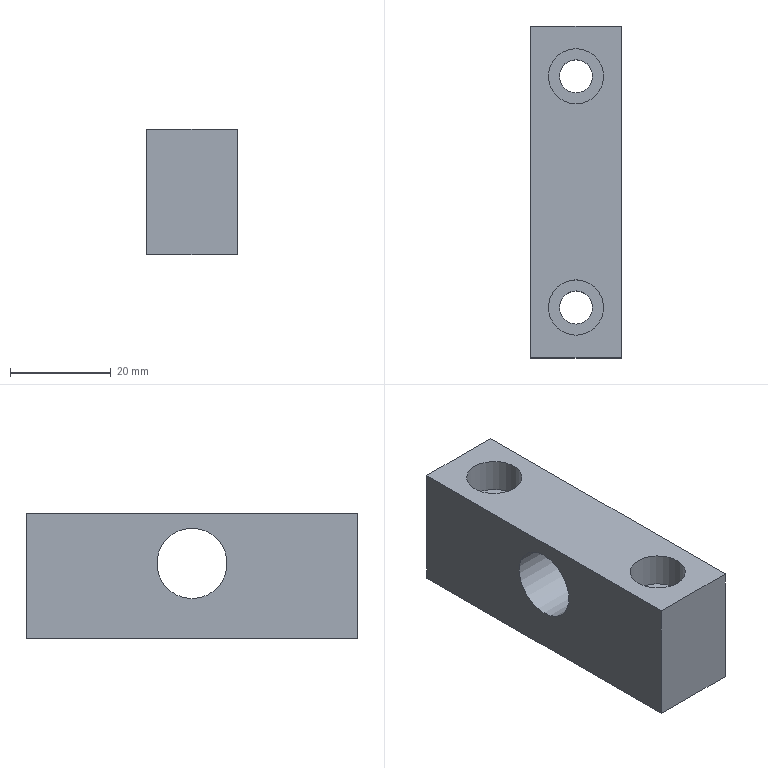Component | NX | FIXED_BLOCK | 1 solid | 13 faces | box 18 x 66 x 25 mm | volume 24391 mm3 | plane 8 | cylinder 5 | commonest cylinder face diameters 6.6 x2 11 x2 14 x1
STEP:
#1=CARTESIAN_POINT('',(0.,0.,0.));
#2=DIRECTION('',(0.,0.,1.));
#3=DIRECTION('',(1.,0.,0.));
#4=AXIS2_PLACEMENT_3D('',#1,#2,#3);
#5=CARTESIAN_POINT('',(-140.,-33.,25.));
#6=VERTEX_POINT('',#5);
#7=CARTESIAN_POINT('',(-122.,-33.,25.));
#8=VERTEX_POINT('',#7);
#9=CARTESIAN_POINT('',(-140.,-33.,25.));
#10=DIRECTION('',(1.,0.,0.));
#11=VECTOR('',#10,1.);
#12=LINE('',#9,#11);
#13=CARTESIAN_POINT('',(-140.,-33.,0.));
#14=DIRECTION('',(0.,-1.,0.));
#15=DIRECTION('',(0.,0.,1.));
#16=AXIS2_PLACEMENT_3D('',#13,#14,#15);
#17=PLANE('',#16);
#18=CARTESIAN_POINT('',(25.,0.));
#19=DIRECTION('',(0.,-1.));
#20=VECTOR('',#19,1.);
#21=LINE('',#18,#20);
#22=(GEOMETRIC_REPRESENTATION_CONTEXT(2)PARAMETRIC_REPRESENTATION_CONTEXT()REPRESENTATION_CONTEXT('',''));
#23=DEFINITIONAL_REPRESENTATION('',(#21),#22);
#24=PCURVE('',#17,#23);
#25=CARTESIAN_POINT('',(-131.,0.,25.));
#26=DIRECTION('',(0.,0.,1.));
#27=DIRECTION('',(0.,1.,0.));
#28=AXIS2_PLACEMENT_3D('',#25,#26,#27);
#29=PLANE('',#28);
#30=CARTESIAN_POINT('',(-33.,9.));
#31=DIRECTION('',(0.,-1.));
#32=VECTOR('',#31,1.);
#33=LINE('',#30,#32);
#34=(GEOMETRIC_REPRESENTATION_CONTEXT(2)PARAMETRIC_REPRESENTATION_CONTEXT()REPRESENTATION_CONTEXT('',''));
#35=DEFINITIONAL_REPRESENTATION('',(#33),#34);
#36=PCURVE('',#29,#35);
#37=SURFACE_CURVE('',#12,(#24,#36),.PCURVE_S1.);
#38=EDGE_CURVE('',#6,#8,#37,.T.);
#39=ORIENTED_EDGE('',*,*,#38,.F.);
#40=CARTESIAN_POINT('',(-140.,-33.,0.));
#41=VERTEX_POINT('',#40);
#42=CARTESIAN_POINT('',(-140.,-33.,0.));
#43=DIRECTION('',(0.,0.,1.));
#44=VECTOR('',#43,1.);
#45=LINE('',#42,#44);
#46=CARTESIAN_POINT('',(0.,0.));
#47=DIRECTION('',(1.,0.));
#48=VECTOR('',#47,1.);
#49=LINE('',#46,#48);
#50=(GEOMETRIC_REPRESENTATION_CONTEXT(2)PARAMETRIC_REPRESENTATION_CONTEXT()REPRESENTATION_CONTEXT('',''));
#51=DEFINITIONAL_REPRESENTATION('',(#49),#50);
#52=PCURVE('',#17,#51);
#53=CARTESIAN_POINT('',(-140.,33.,0.));
#54=DIRECTION('',(-1.,0.,0.));
#55=DIRECTION('',(0.,0.,1.));
#56=AXIS2_PLACEMENT_3D('',#53,#54,#55);
#57=PLANE('',#56);
#58=CARTESIAN_POINT('',(0.,-66.));
#59=DIRECTION('',(1.,0.));
#60=VECTOR('',#59,1.);
#61=LINE('',#58,#60);
#62=(GEOMETRIC_REPRESENTATION_CONTEXT(2)PARAMETRIC_REPRESENTATION_CONTEXT()REPRESENTATION_CONTEXT('',''));
#63=DEFINITIONAL_REPRESENTATION('',(#61),#62);
#64=PCURVE('',#57,#63);
#65=SURFACE_CURVE('',#45,(#52,#64),.PCURVE_S1.);
#66=EDGE_CURVE('',#41,#6,#65,.T.);
#67=ORIENTED_EDGE('',*,*,#66,.F.);
#68=CARTESIAN_POINT('',(-122.,-33.,0.));
#69=VERTEX_POINT('',#68);
#70=CARTESIAN_POINT('',(-140.,-33.,0.));
#71=DIRECTION('',(1.,0.,0.));
#72=VECTOR('',#71,1.);
#73=LINE('',#70,#72);
#74=CARTESIAN_POINT('',(0.,0.));
#75=DIRECTION('',(0.,-1.));
#76=VECTOR('',#75,1.);
#77=LINE('',#74,#76);
#78=(GEOMETRIC_REPRESENTATION_CONTEXT(2)PARAMETRIC_REPRESENTATION_CONTEXT()REPRESENTATION_CONTEXT('',''));
#79=DEFINITIONAL_REPRESENTATION('',(#77),#78);
#80=PCURVE('',#17,#79);
#81=CARTESIAN_POINT('',(-131.,0.,0.));
#82=DIRECTION('',(0.,0.,1.));
#83=DIRECTION('',(0.,1.,0.));
#84=AXIS2_PLACEMENT_3D('',#81,#82,#83);
#85=PLANE('',#84);
#86=CARTESIAN_POINT('',(-33.,9.));
#87=DIRECTION('',(0.,-1.));
#88=VECTOR('',#87,1.);
#89=LINE('',#86,#88);
#90=(GEOMETRIC_REPRESENTATION_CONTEXT(2)PARAMETRIC_REPRESENTATION_CONTEXT()REPRESENTATION_CONTEXT('',''));
#91=DEFINITIONAL_REPRESENTATION('',(#89),#90);
#92=PCURVE('',#85,#91);
#93=SURFACE_CURVE('',#73,(#80,#92),.PCURVE_S1.);
#94=EDGE_CURVE('',#41,#69,#93,.T.);
#95=ORIENTED_EDGE('',*,*,#94,.T.);
#96=CARTESIAN_POINT('',(-122.,-33.,0.));
#97=DIRECTION('',(0.,0.,1.));
#98=VECTOR('',#97,1.);
#99=LINE('',#96,#98);
#100=CARTESIAN_POINT('',(0.,-18.));
#101=DIRECTION('',(1.,0.));
#102=VECTOR('',#101,1.);
#103=LINE('',#100,#102);
#104=(GEOMETRIC_REPRESENTATION_CONTEXT(2)PARAMETRIC_REPRESENTATION_CONTEXT()REPRESENTATION_CONTEXT('',''));
#105=DEFINITIONAL_REPRESENTATION('',(#103),#104);
#106=PCURVE('',#17,#105);
#107=CARTESIAN_POINT('',(-122.,-33.,0.));
#108=DIRECTION('',(1.,0.,0.));
#109=DIRECTION('',(0.,0.,-1.));
#110=AXIS2_PLACEMENT_3D('',#107,#108,#109);
#111=PLANE('',#110);
#112=CARTESIAN_POINT('',(0.,0.));
#113=DIRECTION('',(-1.,0.));
#114=VECTOR('',#113,1.);
#115=LINE('',#112,#114);
#116=(GEOMETRIC_REPRESENTATION_CONTEXT(2)PARAMETRIC_REPRESENTATION_CONTEXT()REPRESENTATION_CONTEXT('',''));
#117=DEFINITIONAL_REPRESENTATION('',(#115),#116);
#118=PCURVE('',#111,#117);
#119=SURFACE_CURVE('',#99,(#106,#118),.PCURVE_S1.);
#120=EDGE_CURVE('',#69,#8,#119,.T.);
#121=ORIENTED_EDGE('',*,*,#120,.T.);
#122=EDGE_LOOP('',(#39,#67,#95,#121));
#123=FACE_BOUND('',#122,.T.);
#124=ADVANCED_FACE('',(#123),#17,.T.);
#125=CARTESIAN_POINT('',(-122.,0.,8.));
#126=VERTEX_POINT('',#125);
#127=CARTESIAN_POINT('',(-122.,0.,15.));
#128=DIRECTION('',(1.,0.,0.));
#129=DIRECTION('',(0.,0.,-1.));
#130=AXIS2_PLACEMENT_3D('',#127,#128,#129);
#131=CIRCLE('',#130,7.);
#132=CARTESIAN_POINT('',(-15.,33.));
#133=DIRECTION('',(1.,0.));
#134=AXIS2_PLACEMENT_2D('',#132,#133);
#135=CIRCLE('',#134,7.);
#136=(GEOMETRIC_REPRESENTATION_CONTEXT(2)PARAMETRIC_REPRESENTATION_CONTEXT()REPRESENTATION_CONTEXT('',''));
#137=DEFINITIONAL_REPRESENTATION('',(#135),#136);
#138=PCURVE('',#111,#137);
#139=CARTESIAN_POINT('',(-121.,0.,15.));
#140=DIRECTION('',(-1.,0.,0.));
#141=DIRECTION('',(0.,1.,0.));
#142=AXIS2_PLACEMENT_3D('',#139,#140,#141);
#143=CYLINDRICAL_SURFACE('',#142,7.);
#144=CARTESIAN_POINT('',(7.854,1.));
#145=DIRECTION('',(-1.,0.));
#146=VECTOR('',#145,1.);
#147=LINE('',#144,#146);
#148=(GEOMETRIC_REPRESENTATION_CONTEXT(2)PARAMETRIC_REPRESENTATION_CONTEXT()REPRESENTATION_CONTEXT('',''));
#149=DEFINITIONAL_REPRESENTATION('',(#147),#148);
#150=PCURVE('',#143,#149);
#151=SURFACE_CURVE('',#131,(#138,#150),.PCURVE_S1.);
#152=EDGE_CURVE('',#126,#126,#151,.T.);
#153=ORIENTED_EDGE('',*,*,#152,.F.);
#154=EDGE_LOOP('',(#153));
#155=FACE_BOUND('',#154,.T.);
#156=CARTESIAN_POINT('',(-122.,33.,25.));
#157=VERTEX_POINT('',#156);
#158=CARTESIAN_POINT('',(-122.,-33.,25.));
#159=DIRECTION('',(0.,1.,0.));
#160=VECTOR('',#159,1.);
#161=LINE('',#158,#160);
#162=CARTESIAN_POINT('',(-25.,0.));
#163=DIRECTION('',(0.,1.));
#164=VECTOR('',#163,1.);
#165=LINE('',#162,#164);
#166=(GEOMETRIC_REPRESENTATION_CONTEXT(2)PARAMETRIC_REPRESENTATION_CONTEXT()REPRESENTATION_CONTEXT('',''));
#167=DEFINITIONAL_REPRESENTATION('',(#165),#166);
#168=PCURVE('',#111,#167);
#169=CARTESIAN_POINT('',(-33.,-9.));
#170=DIRECTION('',(1.,0.));
#171=VECTOR('',#170,1.);
#172=LINE('',#169,#171);
#173=(GEOMETRIC_REPRESENTATION_CONTEXT(2)PARAMETRIC_REPRESENTATION_CONTEXT()REPRESENTATION_CONTEXT('',''));
#174=DEFINITIONAL_REPRESENTATION('',(#172),#173);
#175=PCURVE('',#29,#174);
#176=SURFACE_CURVE('',#161,(#168,#175),.PCURVE_S1.);
#177=EDGE_CURVE('',#8,#157,#176,.T.);
#178=ORIENTED_EDGE('',*,*,#177,.F.);
#179=ORIENTED_EDGE('',*,*,#120,.F.);
#180=CARTESIAN_POINT('',(-122.,33.,0.));
#181=VERTEX_POINT('',#180);
#182=CARTESIAN_POINT('',(-122.,-33.,0.));
#183=DIRECTION('',(0.,1.,0.));
#184=VECTOR('',#183,1.);
#185=LINE('',#182,#184);
#186=CARTESIAN_POINT('',(0.,0.));
#187=DIRECTION('',(0.,1.));
#188=VECTOR('',#187,1.);
#189=LINE('',#186,#188);
#190=(GEOMETRIC_REPRESENTATION_CONTEXT(2)PARAMETRIC_REPRESENTATION_CONTEXT()REPRESENTATION_CONTEXT('',''));
#191=DEFINITIONAL_REPRESENTATION('',(#189),#190);
#192=PCURVE('',#111,#191);
#193=CARTESIAN_POINT('',(-33.,-9.));
#194=DIRECTION('',(1.,0.));
#195=VECTOR('',#194,1.);
#196=LINE('',#193,#195);
#197=(GEOMETRIC_REPRESENTATION_CONTEXT(2)PARAMETRIC_REPRESENTATION_CONTEXT()REPRESENTATION_CONTEXT('',''));
#198=DEFINITIONAL_REPRESENTATION('',(#196),#197);
#199=PCURVE('',#85,#198);
#200=SURFACE_CURVE('',#185,(#192,#199),.PCURVE_S1.);
#201=EDGE_CURVE('',#69,#181,#200,.T.);
#202=ORIENTED_EDGE('',*,*,#201,.T.);
#203=CARTESIAN_POINT('',(-122.,33.,0.));
#204=DIRECTION('',(0.,0.,1.));
#205=VECTOR('',#204,1.);
#206=LINE('',#203,#205);
#207=CARTESIAN_POINT('',(0.,66.));
#208=DIRECTION('',(-1.,0.));
#209=VECTOR('',#208,1.);
#210=LINE('',#207,#209);
#211=(GEOMETRIC_REPRESENTATION_CONTEXT(2)PARAMETRIC_REPRESENTATION_CONTEXT()REPRESENTATION_CONTEXT('',''));
#212=DEFINITIONAL_REPRESENTATION('',(#210),#211);
#213=PCURVE('',#111,#212);
#214=CARTESIAN_POINT('',(-122.,33.,0.));
#215=DIRECTION('',(0.,1.,0.));
#216=DIRECTION('',(0.,0.,-1.));
#217=AXIS2_PLACEMENT_3D('',#214,#215,#216);
#218=PLANE('',#217);
#219=CARTESIAN_POINT('',(0.,0.));
#220=DIRECTION('',(-1.,0.));
#221=VECTOR('',#220,1.);
#222=LINE('',#219,#221);
#223=(GEOMETRIC_REPRESENTATION_CONTEXT(2)PARAMETRIC_REPRESENTATION_CONTEXT()REPRESENTATION_CONTEXT('',''));
#224=DEFINITIONAL_REPRESENTATION('',(#222),#223);
#225=PCURVE('',#218,#224);
#226=SURFACE_CURVE('',#206,(#213,#225),.PCURVE_S1.);
#227=EDGE_CURVE('',#181,#157,#226,.T.);
#228=ORIENTED_EDGE('',*,*,#227,.T.);
#229=EDGE_LOOP('',(#178,#179,#202,#228));
#230=FACE_BOUND('',#229,.T.);
#231=ADVANCED_FACE('',(#155,#230),#111,.T.);
#232=CARTESIAN_POINT('',(-140.,33.,25.));
#233=VERTEX_POINT('',#232);
#234=CARTESIAN_POINT('',(-122.,33.,25.));
#235=DIRECTION('',(-1.,0.,0.));
#236=VECTOR('',#235,1.);
#237=LINE('',#234,#236);
#238=CARTESIAN_POINT('',(-25.,0.));
#239=DIRECTION('',(0.,1.));
#240=VECTOR('',#239,1.);
#241=LINE('',#238,#240);
#242=(GEOMETRIC_REPRESENTATION_CONTEXT(2)PARAMETRIC_REPRESENTATION_CONTEXT()REPRESENTATION_CONTEXT('',''));
#243=DEFINITIONAL_REPRESENTATION('',(#241),#242);
#244=PCURVE('',#218,#243);
#245=CARTESIAN_POINT('',(33.,-9.));
#246=DIRECTION('',(0.,1.));
#247=VECTOR('',#246,1.);
#248=LINE('',#245,#247);
#249=(GEOMETRIC_REPRESENTATION_CONTEXT(2)PARAMETRIC_REPRESENTATION_CONTEXT()REPRESENTATION_CONTEXT('',''));
#250=DEFINITIONAL_REPRESENTATION('',(#248),#249);
#251=PCURVE('',#29,#250);
#252=SURFACE_CURVE('',#237,(#244,#251),.PCURVE_S1.);
#253=EDGE_CURVE('',#157,#233,#252,.T.);
#254=ORIENTED_EDGE('',*,*,#253,.F.);
#255=ORIENTED_EDGE('',*,*,#227,.F.);
#256=CARTESIAN_POINT('',(-140.,33.,0.));
#257=VERTEX_POINT('',#256);
#258=CARTESIAN_POINT('',(-122.,33.,0.));
#259=DIRECTION('',(-1.,0.,0.));
#260=VECTOR('',#259,1.);
#261=LINE('',#258,#260);
#262=CARTESIAN_POINT('',(0.,0.));
#263=DIRECTION('',(0.,1.));
#264=VECTOR('',#263,1.);
#265=LINE('',#262,#264);
#266=(GEOMETRIC_REPRESENTATION_CONTEXT(2)PARAMETRIC_REPRESENTATION_CONTEXT()REPRESENTATION_CONTEXT('',''));
#267=DEFINITIONAL_REPRESENTATION('',(#265),#266);
#268=PCURVE('',#218,#267);
#269=CARTESIAN_POINT('',(33.,-9.));
#270=DIRECTION('',(0.,1.));
#271=VECTOR('',#270,1.);
#272=LINE('',#269,#271);
#273=(GEOMETRIC_REPRESENTATION_CONTEXT(2)PARAMETRIC_REPRESENTATION_CONTEXT()REPRESENTATION_CONTEXT('',''));
#274=DEFINITIONAL_REPRESENTATION('',(#272),#273);
#275=PCURVE('',#85,#274);
#276=SURFACE_CURVE('',#261,(#268,#275),.PCURVE_S1.);
#277=EDGE_CURVE('',#181,#257,#276,.T.);
#278=ORIENTED_EDGE('',*,*,#277,.T.);
#279=CARTESIAN_POINT('',(-140.,33.,0.));
#280=DIRECTION('',(0.,0.,1.));
#281=VECTOR('',#280,1.);
#282=LINE('',#279,#281);
#283=CARTESIAN_POINT('',(0.,18.));
#284=DIRECTION('',(-1.,0.));
#285=VECTOR('',#284,1.);
#286=LINE('',#283,#285);
#287=(GEOMETRIC_REPRESENTATION_CONTEXT(2)PARAMETRIC_REPRESENTATION_CONTEXT()REPRESENTATION_CONTEXT('',''));
#288=DEFINITIONAL_REPRESENTATION('',(#286),#287);
#289=PCURVE('',#218,#288);
#290=CARTESIAN_POINT('',(0.,0.));
#291=DIRECTION('',(1.,0.));
#292=VECTOR('',#291,1.);
#293=LINE('',#290,#292);
#294=(GEOMETRIC_REPRESENTATION_CONTEXT(2)PARAMETRIC_REPRESENTATION_CONTEXT()REPRESENTATION_CONTEXT('',''));
#295=DEFINITIONAL_REPRESENTATION('',(#293),#294);
#296=PCURVE('',#57,#295);
#297=SURFACE_CURVE('',#282,(#289,#296),.PCURVE_S1.);
#298=EDGE_CURVE('',#257,#233,#297,.T.);
#299=ORIENTED_EDGE('',*,*,#298,.T.);
#300=EDGE_LOOP('',(#254,#255,#278,#299));
#301=FACE_BOUND('',#300,.T.);
#302=ADVANCED_FACE('',(#301),#218,.T.);
#303=CARTESIAN_POINT('',(-140.,0.,22.));
#304=VERTEX_POINT('',#303);
#305=CARTESIAN_POINT('',(-140.,0.,8.));
#306=VERTEX_POINT('',#305);
#307=CARTESIAN_POINT('',(-140.,0.,15.));
#308=DIRECTION('',(-1.,0.,0.));
#309=DIRECTION('',(0.,0.,1.));
#310=AXIS2_PLACEMENT_3D('',#307,#308,#309);
#311=CIRCLE('',#310,7.);
#312=CARTESIAN_POINT('',(15.,-33.));
#313=DIRECTION('',(1.,0.));
#314=AXIS2_PLACEMENT_2D('',#312,#313);
#315=CIRCLE('',#314,7.);
#316=(GEOMETRIC_REPRESENTATION_CONTEXT(2)PARAMETRIC_REPRESENTATION_CONTEXT()REPRESENTATION_CONTEXT('',''));
#317=DEFINITIONAL_REPRESENTATION('',(#315),#316);
#318=PCURVE('',#57,#317);
#319=CARTESIAN_POINT('',(4.712,19.));
#320=DIRECTION('',(1.,0.));
#321=VECTOR('',#320,1.);
#322=LINE('',#319,#321);
#323=(GEOMETRIC_REPRESENTATION_CONTEXT(2)PARAMETRIC_REPRESENTATION_CONTEXT()REPRESENTATION_CONTEXT('',''));
#324=DEFINITIONAL_REPRESENTATION('',(#322),#323);
#325=PCURVE('',#143,#324);
#326=SURFACE_CURVE('',#311,(#318,#325),.PCURVE_S1.);
#327=EDGE_CURVE('',#304,#306,#326,.T.);
#328=ORIENTED_EDGE('',*,*,#327,.F.);
#329=CARTESIAN_POINT('',(-140.,0.,15.));
#330=DIRECTION('',(-1.,0.,0.));
#331=DIRECTION('',(0.,0.,1.));
#332=AXIS2_PLACEMENT_3D('',#329,#330,#331);
#333=CIRCLE('',#332,7.);
#334=CARTESIAN_POINT('',(15.,-33.));
#335=DIRECTION('',(1.,0.));
#336=AXIS2_PLACEMENT_2D('',#334,#335);
#337=CIRCLE('',#336,7.);
#338=(GEOMETRIC_REPRESENTATION_CONTEXT(2)PARAMETRIC_REPRESENTATION_CONTEXT()REPRESENTATION_CONTEXT('',''));
#339=DEFINITIONAL_REPRESENTATION('',(#337),#338);
#340=PCURVE('',#57,#339);
#341=CARTESIAN_POINT('',(-1.571,19.));
#342=DIRECTION('',(1.,0.));
#343=VECTOR('',#342,1.);
#344=LINE('',#341,#343);
#345=(GEOMETRIC_REPRESENTATION_CONTEXT(2)PARAMETRIC_REPRESENTATION_CONTEXT()REPRESENTATION_CONTEXT('',''));
#346=DEFINITIONAL_REPRESENTATION('',(#344),#345);
#347=PCURVE('',#143,#346);
#348=SURFACE_CURVE('',#333,(#340,#347),.PCURVE_S1.);
#349=EDGE_CURVE('',#306,#304,#348,.T.);
#350=ORIENTED_EDGE('',*,*,#349,.F.);
#351=EDGE_LOOP('',(#328,#350));
#352=FACE_BOUND('',#351,.T.);
#353=CARTESIAN_POINT('',(-140.,33.,25.));
#354=DIRECTION('',(0.,-1.,0.));
#355=VECTOR('',#354,1.);
#356=LINE('',#353,#355);
#357=CARTESIAN_POINT('',(25.,0.));
#358=DIRECTION('',(0.,-1.));
#359=VECTOR('',#358,1.);
#360=LINE('',#357,#359);
#361=(GEOMETRIC_REPRESENTATION_CONTEXT(2)PARAMETRIC_REPRESENTATION_CONTEXT()REPRESENTATION_CONTEXT('',''));
#362=DEFINITIONAL_REPRESENTATION('',(#360),#361);
#363=PCURVE('',#57,#362);
#364=CARTESIAN_POINT('',(33.,9.));
#365=DIRECTION('',(-1.,0.));
#366=VECTOR('',#365,1.);
#367=LINE('',#364,#366);
#368=(GEOMETRIC_REPRESENTATION_CONTEXT(2)PARAMETRIC_REPRESENTATION_CONTEXT()REPRESENTATION_CONTEXT('',''));
#369=DEFINITIONAL_REPRESENTATION('',(#367),#368);
#370=PCURVE('',#29,#369);
#371=SURFACE_CURVE('',#356,(#363,#370),.PCURVE_S1.);
#372=EDGE_CURVE('',#233,#6,#371,.T.);
#373=ORIENTED_EDGE('',*,*,#372,.F.);
#374=ORIENTED_EDGE('',*,*,#298,.F.);
#375=CARTESIAN_POINT('',(-140.,33.,0.));
#376=DIRECTION('',(0.,-1.,0.));
#377=VECTOR('',#376,1.);
#378=LINE('',#375,#377);
#379=CARTESIAN_POINT('',(0.,0.));
#380=DIRECTION('',(0.,-1.));
#381=VECTOR('',#380,1.);
#382=LINE('',#379,#381);
#383=(GEOMETRIC_REPRESENTATION_CONTEXT(2)PARAMETRIC_REPRESENTATION_CONTEXT()REPRESENTATION_CONTEXT('',''));
#384=DEFINITIONAL_REPRESENTATION('',(#382),#383);
#385=PCURVE('',#57,#384);
#386=CARTESIAN_POINT('',(33.,9.));
#387=DIRECTION('',(-1.,0.));
#388=VECTOR('',#387,1.);
#389=LINE('',#386,#388);
#390=(GEOMETRIC_REPRESENTATION_CONTEXT(2)PARAMETRIC_REPRESENTATION_CONTEXT()REPRESENTATION_CONTEXT('',''));
#391=DEFINITIONAL_REPRESENTATION('',(#389),#390);
#392=PCURVE('',#85,#391);
#393=SURFACE_CURVE('',#378,(#385,#392),.PCURVE_S1.);
#394=EDGE_CURVE('',#257,#41,#393,.T.);
#395=ORIENTED_EDGE('',*,*,#394,.T.);
#396=ORIENTED_EDGE('',*,*,#66,.T.);
#397=EDGE_LOOP('',(#373,#374,#395,#396));
#398=FACE_BOUND('',#397,.T.);
#399=ADVANCED_FACE('',(#352,#398),#57,.T.);
#400=CARTESIAN_POINT('',(-131.,26.3,0.));
#401=VERTEX_POINT('',#400);
#402=CARTESIAN_POINT('',(-131.,19.7,0.));
#403=VERTEX_POINT('',#402);
#404=CARTESIAN_POINT('',(-131.,23.,0.));
#405=DIRECTION('',(0.,0.,1.));
#406=DIRECTION('',(0.,1.,0.));
#407=AXIS2_PLACEMENT_3D('',#404,#405,#406);
#408=CIRCLE('',#407,3.3);
#409=CARTESIAN_POINT('',(23.,0.));
#410=DIRECTION('',(1.,0.));
#411=AXIS2_PLACEMENT_2D('',#409,#410);
#412=CIRCLE('',#411,3.3);
#413=(GEOMETRIC_REPRESENTATION_CONTEXT(2)PARAMETRIC_REPRESENTATION_CONTEXT()REPRESENTATION_CONTEXT('',''));
#414=DEFINITIONAL_REPRESENTATION('',(#412),#413);
#415=PCURVE('',#85,#414);
#416=CARTESIAN_POINT('',(-131.,23.,-20.299));
#417=DIRECTION('',(0.,0.,-1.));
#418=DIRECTION('',(0.,-1.,0.));
#419=AXIS2_PLACEMENT_3D('',#416,#417,#418);
#420=CYLINDRICAL_SURFACE('',#419,3.3);
#421=CARTESIAN_POINT('',(3.142,-20.299));
#422=DIRECTION('',(-1.,0.));
#423=VECTOR('',#422,1.);
#424=LINE('',#421,#423);
#425=(GEOMETRIC_REPRESENTATION_CONTEXT(2)PARAMETRIC_REPRESENTATION_CONTEXT()REPRESENTATION_CONTEXT('',''));
#426=DEFINITIONAL_REPRESENTATION('',(#424),#425);
#427=PCURVE('',#420,#426);
#428=SURFACE_CURVE('',#408,(#415,#427),.PCURVE_S1.);
#429=EDGE_CURVE('',#401,#403,#428,.T.);
#430=ORIENTED_EDGE('',*,*,#429,.T.);
#431=CARTESIAN_POINT('',(-131.,23.,0.));
#432=DIRECTION('',(0.,0.,1.));
#433=DIRECTION('',(0.,1.,0.));
#434=AXIS2_PLACEMENT_3D('',#431,#432,#433);
#435=CIRCLE('',#434,3.3);
#436=CARTESIAN_POINT('',(23.,0.));
#437=DIRECTION('',(1.,0.));
#438=AXIS2_PLACEMENT_2D('',#436,#437);
#439=CIRCLE('',#438,3.3);
#440=(GEOMETRIC_REPRESENTATION_CONTEXT(2)PARAMETRIC_REPRESENTATION_CONTEXT()REPRESENTATION_CONTEXT('',''));
#441=DEFINITIONAL_REPRESENTATION('',(#439),#440);
#442=PCURVE('',#85,#441);
#443=CARTESIAN_POINT('',(9.425,-20.299));
#444=DIRECTION('',(-1.,0.));
#445=VECTOR('',#444,1.);
#446=LINE('',#443,#445);
#447=(GEOMETRIC_REPRESENTATION_CONTEXT(2)PARAMETRIC_REPRESENTATION_CONTEXT()REPRESENTATION_CONTEXT('',''));
#448=DEFINITIONAL_REPRESENTATION('',(#446),#447);
#449=PCURVE('',#420,#448);
#450=SURFACE_CURVE('',#435,(#442,#449),.PCURVE_S1.);
#451=EDGE_CURVE('',#403,#401,#450,.T.);
#452=ORIENTED_EDGE('',*,*,#451,.T.);
#453=EDGE_LOOP('',(#430,#452));
#454=FACE_BOUND('',#453,.T.);
#455=CARTESIAN_POINT('',(-131.,-19.7,0.));
#456=VERTEX_POINT('',#455);
#457=CARTESIAN_POINT('',(-131.,-26.3,0.));
#458=VERTEX_POINT('',#457);
#459=CARTESIAN_POINT('',(-131.,-23.,0.));
#460=DIRECTION('',(0.,0.,1.));
#461=DIRECTION('',(0.,1.,0.));
#462=AXIS2_PLACEMENT_3D('',#459,#460,#461);
#463=CIRCLE('',#462,3.3);
#464=CARTESIAN_POINT('',(-23.,0.));
#465=DIRECTION('',(1.,0.));
#466=AXIS2_PLACEMENT_2D('',#464,#465);
#467=CIRCLE('',#466,3.3);
#468=(GEOMETRIC_REPRESENTATION_CONTEXT(2)PARAMETRIC_REPRESENTATION_CONTEXT()REPRESENTATION_CONTEXT('',''));
#469=DEFINITIONAL_REPRESENTATION('',(#467),#468);
#470=PCURVE('',#85,#469);
#471=CARTESIAN_POINT('',(-131.,-23.,-20.299));
#472=DIRECTION('',(0.,0.,-1.));
#473=DIRECTION('',(0.,-1.,0.));
#474=AXIS2_PLACEMENT_3D('',#471,#472,#473);
#475=CYLINDRICAL_SURFACE('',#474,3.3);
#476=CARTESIAN_POINT('',(3.142,-20.299));
#477=DIRECTION('',(-1.,0.));
#478=VECTOR('',#477,1.);
#479=LINE('',#476,#478);
#480=(GEOMETRIC_REPRESENTATION_CONTEXT(2)PARAMETRIC_REPRESENTATION_CONTEXT()REPRESENTATION_CONTEXT('',''));
#481=DEFINITIONAL_REPRESENTATION('',(#479),#480);
#482=PCURVE('',#475,#481);
#483=SURFACE_CURVE('',#463,(#470,#482),.PCURVE_S1.);
#484=EDGE_CURVE('',#456,#458,#483,.T.);
#485=ORIENTED_EDGE('',*,*,#484,.T.);
#486=CARTESIAN_POINT('',(-131.,-23.,0.));
#487=DIRECTION('',(0.,0.,1.));
#488=DIRECTION('',(0.,1.,0.));
#489=AXIS2_PLACEMENT_3D('',#486,#487,#488);
#490=CIRCLE('',#489,3.3);
#491=CARTESIAN_POINT('',(-23.,0.));
#492=DIRECTION('',(1.,0.));
#493=AXIS2_PLACEMENT_2D('',#491,#492);
#494=CIRCLE('',#493,3.3);
#495=(GEOMETRIC_REPRESENTATION_CONTEXT(2)PARAMETRIC_REPRESENTATION_CONTEXT()REPRESENTATION_CONTEXT('',''));
#496=DEFINITIONAL_REPRESENTATION('',(#494),#495);
#497=PCURVE('',#85,#496);
#498=CARTESIAN_POINT('',(9.425,-20.299));
#499=DIRECTION('',(-1.,0.));
#500=VECTOR('',#499,1.);
#501=LINE('',#498,#500);
#502=(GEOMETRIC_REPRESENTATION_CONTEXT(2)PARAMETRIC_REPRESENTATION_CONTEXT()REPRESENTATION_CONTEXT('',''));
#503=DEFINITIONAL_REPRESENTATION('',(#501),#502);
#504=PCURVE('',#475,#503);
#505=SURFACE_CURVE('',#490,(#497,#504),.PCURVE_S1.);
#506=EDGE_CURVE('',#458,#456,#505,.T.);
#507=ORIENTED_EDGE('',*,*,#506,.T.);
#508=EDGE_LOOP('',(#485,#507));
#509=FACE_BOUND('',#508,.T.);
#510=ORIENTED_EDGE('',*,*,#94,.F.);
#511=ORIENTED_EDGE('',*,*,#394,.F.);
#512=ORIENTED_EDGE('',*,*,#277,.F.);
#513=ORIENTED_EDGE('',*,*,#201,.F.);
#514=EDGE_LOOP('',(#510,#511,#512,#513));
#515=FACE_BOUND('',#514,.T.);
#516=ADVANCED_FACE('',(#454,#509,#515),#85,.F.);
#517=CARTESIAN_POINT('',(-131.,17.5,25.));
#518=VERTEX_POINT('',#517);
#519=CARTESIAN_POINT('',(-131.,23.,25.));
#520=DIRECTION('',(0.,0.,-1.));
#521=DIRECTION('',(0.,-1.,0.));
#522=AXIS2_PLACEMENT_3D('',#519,#520,#521);
#523=CIRCLE('',#522,5.5);
#524=CARTESIAN_POINT('',(17.5,0.));
#525=CARTESIAN_POINT('',(17.5,9.526));
#526=CARTESIAN_POINT('',(25.75,4.763));
#527=CARTESIAN_POINT('',(34.,0.));
#528=CARTESIAN_POINT('',(25.75,-4.763));
#529=CARTESIAN_POINT('',(17.5,-9.526));
#530=CARTESIAN_POINT('',(17.5,0.));
#531=(BOUNDED_CURVE()B_SPLINE_CURVE(2,(#524,#525,#526,#527,#528,#529,#530),.UNSPECIFIED.,.T.,.F.)B_SPLINE_CURVE_WITH_KNOTS((1,2,2,2,2,1),(-2.094,0.,2.094,4.189,6.283,8.378),.UNSPECIFIED.)CURVE()GEOMETRIC_REPRESENTATION_ITEM()RATIONAL_B_SPLINE_CURVE((1.,0.5,1.,0.5,1.,0.5,1.))REPRESENTATION_ITEM(''));
#532=(GEOMETRIC_REPRESENTATION_CONTEXT(2)PARAMETRIC_REPRESENTATION_CONTEXT()REPRESENTATION_CONTEXT('',''));
#533=DEFINITIONAL_REPRESENTATION('',(#531),#532);
#534=PCURVE('',#29,#533);
#535=CARTESIAN_POINT('',(-131.,23.,25.));
#536=DIRECTION('',(0.,0.,-1.));
#537=DIRECTION('',(0.,-1.,0.));
#538=AXIS2_PLACEMENT_3D('',#535,#536,#537);
#539=CYLINDRICAL_SURFACE('',#538,5.5);
#540=CARTESIAN_POINT('',(0.,0.));
#541=DIRECTION('',(1.,0.));
#542=VECTOR('',#541,1.);
#543=LINE('',#540,#542);
#544=(GEOMETRIC_REPRESENTATION_CONTEXT(2)PARAMETRIC_REPRESENTATION_CONTEXT()REPRESENTATION_CONTEXT('',''));
#545=DEFINITIONAL_REPRESENTATION('',(#543),#544);
#546=PCURVE('',#539,#545);
#547=SURFACE_CURVE('',#523,(#534,#546),.PCURVE_S1.);
#548=EDGE_CURVE('',#518,#518,#547,.T.);
#549=ORIENTED_EDGE('',*,*,#548,.T.);
#550=EDGE_LOOP('',(#549));
#551=FACE_BOUND('',#550,.T.);
#552=CARTESIAN_POINT('',(-131.,-28.5,25.));
#553=VERTEX_POINT('',#552);
#554=CARTESIAN_POINT('',(-131.,-23.,25.));
#555=DIRECTION('',(0.,0.,-1.));
#556=DIRECTION('',(0.,-1.,0.));
#557=AXIS2_PLACEMENT_3D('',#554,#555,#556);
#558=CIRCLE('',#557,5.5);
#559=CARTESIAN_POINT('',(-28.5,0.));
#560=CARTESIAN_POINT('',(-28.5,9.526));
#561=CARTESIAN_POINT('',(-20.25,4.763));
#562=CARTESIAN_POINT('',(-12.,0.));
#563=CARTESIAN_POINT('',(-20.25,-4.763));
#564=CARTESIAN_POINT('',(-28.5,-9.526));
#565=CARTESIAN_POINT('',(-28.5,0.));
#566=(BOUNDED_CURVE()B_SPLINE_CURVE(2,(#559,#560,#561,#562,#563,#564,#565),.UNSPECIFIED.,.T.,.F.)B_SPLINE_CURVE_WITH_KNOTS((1,2,2,2,2,1),(-2.094,0.,2.094,4.189,6.283,8.378),.UNSPECIFIED.)CURVE()GEOMETRIC_REPRESENTATION_ITEM()RATIONAL_B_SPLINE_CURVE((1.,0.5,1.,0.5,1.,0.5,1.))REPRESENTATION_ITEM(''));
#567=(GEOMETRIC_REPRESENTATION_CONTEXT(2)PARAMETRIC_REPRESENTATION_CONTEXT()REPRESENTATION_CONTEXT('',''));
#568=DEFINITIONAL_REPRESENTATION('',(#566),#567);
#569=PCURVE('',#29,#568);
#570=CARTESIAN_POINT('',(-131.,-23.,25.));
#571=DIRECTION('',(0.,0.,-1.));
#572=DIRECTION('',(0.,-1.,0.));
#573=AXIS2_PLACEMENT_3D('',#570,#571,#572);
#574=CYLINDRICAL_SURFACE('',#573,5.5);
#575=CARTESIAN_POINT('',(0.,0.));
#576=DIRECTION('',(1.,0.));
#577=VECTOR('',#576,1.);
#578=LINE('',#575,#577);
#579=(GEOMETRIC_REPRESENTATION_CONTEXT(2)PARAMETRIC_REPRESENTATION_CONTEXT()REPRESENTATION_CONTEXT('',''));
#580=DEFINITIONAL_REPRESENTATION('',(#578),#579);
#581=PCURVE('',#574,#580);
#582=SURFACE_CURVE('',#558,(#569,#581),.PCURVE_S1.);
#583=EDGE_CURVE('',#553,#553,#582,.T.);
#584=ORIENTED_EDGE('',*,*,#583,.T.);
#585=EDGE_LOOP('',(#584));
#586=FACE_BOUND('',#585,.T.);
#587=ORIENTED_EDGE('',*,*,#38,.T.);
#588=ORIENTED_EDGE('',*,*,#177,.T.);
#589=ORIENTED_EDGE('',*,*,#253,.T.);
#590=ORIENTED_EDGE('',*,*,#372,.T.);
#591=EDGE_LOOP('',(#587,#588,#589,#590));
#592=FACE_BOUND('',#591,.T.);
#593=ADVANCED_FACE('',(#551,#586,#592),#29,.T.);
#594=CARTESIAN_POINT('',(-131.,-26.3,18.2));
#595=VERTEX_POINT('',#594);
#596=CARTESIAN_POINT('',(-131.,-23.,18.2));
#597=DIRECTION('',(0.,0.,1.));
#598=DIRECTION('',(0.,-1.,0.));
#599=AXIS2_PLACEMENT_3D('',#596,#597,#598);
#600=CIRCLE('',#599,3.3);
#601=CARTESIAN_POINT('',(6.283,-38.499));
#602=DIRECTION('',(-1.,0.));
#603=VECTOR('',#602,1.);
#604=LINE('',#601,#603);
#605=(GEOMETRIC_REPRESENTATION_CONTEXT(2)PARAMETRIC_REPRESENTATION_CONTEXT()REPRESENTATION_CONTEXT('',''));
#606=DEFINITIONAL_REPRESENTATION('',(#604),#605);
#607=PCURVE('',#475,#606);
#608=CARTESIAN_POINT('',(-131.,-23.,18.2));
#609=DIRECTION('',(0.,0.,-1.));
#610=DIRECTION('',(0.,-1.,0.));
#611=AXIS2_PLACEMENT_3D('',#608,#609,#610);
#612=PLANE('',#611);
#613=CARTESIAN_POINT('',(3.3,0.));
#614=CARTESIAN_POINT('',(3.3,-5.716));
#615=CARTESIAN_POINT('',(-1.65,-2.858));
#616=CARTESIAN_POINT('',(-6.6,-0.));
#617=CARTESIAN_POINT('',(-1.65,2.858));
#618=CARTESIAN_POINT('',(3.3,5.716));
#619=CARTESIAN_POINT('',(3.3,0.));
#620=(BOUNDED_CURVE()B_SPLINE_CURVE(2,(#613,#614,#615,#616,#617,#618,#619),.UNSPECIFIED.,.T.,.F.)B_SPLINE_CURVE_WITH_KNOTS((1,2,2,2,2,1),(-2.094,0.,2.094,4.189,6.283,8.378),.UNSPECIFIED.)CURVE()GEOMETRIC_REPRESENTATION_ITEM()RATIONAL_B_SPLINE_CURVE((1.,0.5,1.,0.5,1.,0.5,1.))REPRESENTATION_ITEM(''));
#621=(GEOMETRIC_REPRESENTATION_CONTEXT(2)PARAMETRIC_REPRESENTATION_CONTEXT()REPRESENTATION_CONTEXT('',''));
#622=DEFINITIONAL_REPRESENTATION('',(#620),#621);
#623=PCURVE('',#612,#622);
#624=SURFACE_CURVE('',#600,(#607,#623),.PCURVE_S1.);
#625=EDGE_CURVE('',#595,#595,#624,.T.);
#626=ORIENTED_EDGE('',*,*,#625,.F.);
#627=CARTESIAN_POINT('',(-131.,-26.3,18.2));
#628=CARTESIAN_POINT('',(-131.,-26.3,0.));
#629=B_SPLINE_CURVE_WITH_KNOTS('',1,(#627,#628),.UNSPECIFIED.,.F.,.F.,(2,2),(-38.499,-20.299),.PIECEWISE_BEZIER_KNOTS.);
#630=CARTESIAN_POINT('',(6.283,0.));
#631=DIRECTION('',(0.,1.));
#632=VECTOR('',#631,1.);
#633=LINE('',#630,#632);
#634=(GEOMETRIC_REPRESENTATION_CONTEXT(2)PARAMETRIC_REPRESENTATION_CONTEXT()REPRESENTATION_CONTEXT('',''));
#635=DEFINITIONAL_REPRESENTATION('',(#633),#634);
#636=PCURVE('',#475,#635);
#637=CARTESIAN_POINT('',(0.,0.));
#638=DIRECTION('',(0.,1.));
#639=VECTOR('',#638,1.);
#640=LINE('',#637,#639);
#641=(GEOMETRIC_REPRESENTATION_CONTEXT(2)PARAMETRIC_REPRESENTATION_CONTEXT()REPRESENTATION_CONTEXT('',''));
#642=DEFINITIONAL_REPRESENTATION('',(#640),#641);
#643=PCURVE('',#475,#642);
#644=SEAM_CURVE('',#629,(#636,#643),.PCURVE_S1.);
#645=EDGE_CURVE('',#595,#458,#644,.T.);
#646=ORIENTED_EDGE('',*,*,#645,.T.);
#647=ORIENTED_EDGE('',*,*,#506,.T.);
#648=ORIENTED_EDGE('',*,*,#484,.T.);
#649=ORIENTED_EDGE('',*,*,#645,.F.);
#650=EDGE_LOOP('',(#626,#646,#647,#648,#649));
#651=FACE_BOUND('',#650,.F.);
#652=ADVANCED_FACE('',(#651),#475,.F.);
#653=ORIENTED_EDGE('',*,*,#625,.F.);
#654=EDGE_LOOP('',(#653));
#655=FACE_BOUND('',#654,.T.);
#656=CARTESIAN_POINT('',(-131.,-28.5,18.2));
#657=VERTEX_POINT('',#656);
#658=CARTESIAN_POINT('',(-131.,-23.,18.2));
#659=DIRECTION('',(0.,0.,1.));
#660=DIRECTION('',(0.,-1.,0.));
#661=AXIS2_PLACEMENT_3D('',#658,#659,#660);
#662=CIRCLE('',#661,5.5);
#663=CARTESIAN_POINT('',(5.5,0.));
#664=CARTESIAN_POINT('',(5.5,-9.526));
#665=CARTESIAN_POINT('',(-2.75,-4.763));
#666=CARTESIAN_POINT('',(-11.,-0.));
#667=CARTESIAN_POINT('',(-2.75,4.763));
#668=CARTESIAN_POINT('',(5.5,9.526));
#669=CARTESIAN_POINT('',(5.5,0.));
#670=(BOUNDED_CURVE()B_SPLINE_CURVE(2,(#663,#664,#665,#666,#667,#668,#669),.UNSPECIFIED.,.T.,.F.)B_SPLINE_CURVE_WITH_KNOTS((1,2,2,2,2,1),(-2.094,0.,2.094,4.189,6.283,8.378),.UNSPECIFIED.)CURVE()GEOMETRIC_REPRESENTATION_ITEM()RATIONAL_B_SPLINE_CURVE((1.,0.5,1.,0.5,1.,0.5,1.))REPRESENTATION_ITEM(''));
#671=(GEOMETRIC_REPRESENTATION_CONTEXT(2)PARAMETRIC_REPRESENTATION_CONTEXT()REPRESENTATION_CONTEXT('',''));
#672=DEFINITIONAL_REPRESENTATION('',(#670),#671);
#673=PCURVE('',#612,#672);
#674=CARTESIAN_POINT('',(6.283,6.8));
#675=DIRECTION('',(-1.,0.));
#676=VECTOR('',#675,1.);
#677=LINE('',#674,#676);
#678=(GEOMETRIC_REPRESENTATION_CONTEXT(2)PARAMETRIC_REPRESENTATION_CONTEXT()REPRESENTATION_CONTEXT('',''));
#679=DEFINITIONAL_REPRESENTATION('',(#677),#678);
#680=PCURVE('',#574,#679);
#681=SURFACE_CURVE('',#662,(#673,#680),.PCURVE_S1.);
#682=EDGE_CURVE('',#657,#657,#681,.T.);
#683=ORIENTED_EDGE('',*,*,#682,.T.);
#684=EDGE_LOOP('',(#683));
#685=FACE_BOUND('',#684,.T.);
#686=ADVANCED_FACE('',(#655,#685),#612,.F.);
#687=ORIENTED_EDGE('',*,*,#682,.T.);
#688=CARTESIAN_POINT('',(-131.,-28.5,25.));
#689=CARTESIAN_POINT('',(-131.,-28.5,18.2));
#690=B_SPLINE_CURVE_WITH_KNOTS('',1,(#688,#689),.UNSPECIFIED.,.F.,.F.,(2,2),(0.,6.8),.PIECEWISE_BEZIER_KNOTS.);
#691=CARTESIAN_POINT('',(0.,0.));
#692=DIRECTION('',(0.,1.));
#693=VECTOR('',#692,1.);
#694=LINE('',#691,#693);
#695=(GEOMETRIC_REPRESENTATION_CONTEXT(2)PARAMETRIC_REPRESENTATION_CONTEXT()REPRESENTATION_CONTEXT('',''));
#696=DEFINITIONAL_REPRESENTATION('',(#694),#695);
#697=PCURVE('',#574,#696);
#698=CARTESIAN_POINT('',(6.283,0.));
#699=DIRECTION('',(0.,1.));
#700=VECTOR('',#699,1.);
#701=LINE('',#698,#700);
#702=(GEOMETRIC_REPRESENTATION_CONTEXT(2)PARAMETRIC_REPRESENTATION_CONTEXT()REPRESENTATION_CONTEXT('',''));
#703=DEFINITIONAL_REPRESENTATION('',(#701),#702);
#704=PCURVE('',#574,#703);
#705=SEAM_CURVE('',#690,(#697,#704),.PCURVE_S1.);
#706=EDGE_CURVE('',#553,#657,#705,.T.);
#707=ORIENTED_EDGE('',*,*,#706,.F.);
#708=ORIENTED_EDGE('',*,*,#583,.T.);
#709=ORIENTED_EDGE('',*,*,#706,.T.);
#710=EDGE_LOOP('',(#687,#707,#708,#709));
#711=FACE_BOUND('',#710,.F.);
#712=ADVANCED_FACE('',(#711),#574,.F.);
#713=CARTESIAN_POINT('',(-131.,19.7,18.2));
#714=VERTEX_POINT('',#713);
#715=CARTESIAN_POINT('',(-131.,23.,18.2));
#716=DIRECTION('',(0.,0.,1.));
#717=DIRECTION('',(0.,-1.,0.));
#718=AXIS2_PLACEMENT_3D('',#715,#716,#717);
#719=CIRCLE('',#718,3.3);
#720=CARTESIAN_POINT('',(6.283,-38.499));
#721=DIRECTION('',(-1.,0.));
#722=VECTOR('',#721,1.);
#723=LINE('',#720,#722);
#724=(GEOMETRIC_REPRESENTATION_CONTEXT(2)PARAMETRIC_REPRESENTATION_CONTEXT()REPRESENTATION_CONTEXT('',''));
#725=DEFINITIONAL_REPRESENTATION('',(#723),#724);
#726=PCURVE('',#420,#725);
#727=CARTESIAN_POINT('',(-131.,23.,18.2));
#728=DIRECTION('',(0.,0.,-1.));
#729=DIRECTION('',(0.,-1.,0.));
#730=AXIS2_PLACEMENT_3D('',#727,#728,#729);
#731=PLANE('',#730);
#732=CARTESIAN_POINT('',(3.3,0.));
#733=CARTESIAN_POINT('',(3.3,-5.716));
#734=CARTESIAN_POINT('',(-1.65,-2.858));
#735=CARTESIAN_POINT('',(-6.6,-0.));
#736=CARTESIAN_POINT('',(-1.65,2.858));
#737=CARTESIAN_POINT('',(3.3,5.716));
#738=CARTESIAN_POINT('',(3.3,0.));
#739=(BOUNDED_CURVE()B_SPLINE_CURVE(2,(#732,#733,#734,#735,#736,#737,#738),.UNSPECIFIED.,.T.,.F.)B_SPLINE_CURVE_WITH_KNOTS((1,2,2,2,2,1),(-2.094,0.,2.094,4.189,6.283,8.378),.UNSPECIFIED.)CURVE()GEOMETRIC_REPRESENTATION_ITEM()RATIONAL_B_SPLINE_CURVE((1.,0.5,1.,0.5,1.,0.5,1.))REPRESENTATION_ITEM(''));
#740=(GEOMETRIC_REPRESENTATION_CONTEXT(2)PARAMETRIC_REPRESENTATION_CONTEXT()REPRESENTATION_CONTEXT('',''));
#741=DEFINITIONAL_REPRESENTATION('',(#739),#740);
#742=PCURVE('',#731,#741);
#743=SURFACE_CURVE('',#719,(#726,#742),.PCURVE_S1.);
#744=EDGE_CURVE('',#714,#714,#743,.T.);
#745=ORIENTED_EDGE('',*,*,#744,.F.);
#746=CARTESIAN_POINT('',(-131.,19.7,18.2));
#747=CARTESIAN_POINT('',(-131.,19.7,0.));
#748=B_SPLINE_CURVE_WITH_KNOTS('',1,(#746,#747),.UNSPECIFIED.,.F.,.F.,(2,2),(-38.499,-20.299),.PIECEWISE_BEZIER_KNOTS.);
#749=CARTESIAN_POINT('',(6.283,0.));
#750=DIRECTION('',(0.,1.));
#751=VECTOR('',#750,1.);
#752=LINE('',#749,#751);
#753=(GEOMETRIC_REPRESENTATION_CONTEXT(2)PARAMETRIC_REPRESENTATION_CONTEXT()REPRESENTATION_CONTEXT('',''));
#754=DEFINITIONAL_REPRESENTATION('',(#752),#753);
#755=PCURVE('',#420,#754);
#756=CARTESIAN_POINT('',(0.,0.));
#757=DIRECTION('',(0.,1.));
#758=VECTOR('',#757,1.);
#759=LINE('',#756,#758);
#760=(GEOMETRIC_REPRESENTATION_CONTEXT(2)PARAMETRIC_REPRESENTATION_CONTEXT()REPRESENTATION_CONTEXT('',''));
#761=DEFINITIONAL_REPRESENTATION('',(#759),#760);
#762=PCURVE('',#420,#761);
#763=SEAM_CURVE('',#748,(#755,#762),.PCURVE_S1.);
#764=EDGE_CURVE('',#714,#403,#763,.T.);
#765=ORIENTED_EDGE('',*,*,#764,.T.);
#766=ORIENTED_EDGE('',*,*,#451,.T.);
#767=ORIENTED_EDGE('',*,*,#429,.T.);
#768=ORIENTED_EDGE('',*,*,#764,.F.);
#769=EDGE_LOOP('',(#745,#765,#766,#767,#768));
#770=FACE_BOUND('',#769,.F.);
#771=ADVANCED_FACE('',(#770),#420,.F.);
#772=ORIENTED_EDGE('',*,*,#744,.F.);
#773=EDGE_LOOP('',(#772));
#774=FACE_BOUND('',#773,.T.);
#775=CARTESIAN_POINT('',(-131.,17.5,18.2));
#776=VERTEX_POINT('',#775);
#777=CARTESIAN_POINT('',(-131.,23.,18.2));
#778=DIRECTION('',(0.,0.,1.));
#779=DIRECTION('',(0.,-1.,0.));
#780=AXIS2_PLACEMENT_3D('',#777,#778,#779);
#781=CIRCLE('',#780,5.5);
#782=CARTESIAN_POINT('',(5.5,0.));
#783=CARTESIAN_POINT('',(5.5,-9.526));
#784=CARTESIAN_POINT('',(-2.75,-4.763));
#785=CARTESIAN_POINT('',(-11.,-0.));
#786=CARTESIAN_POINT('',(-2.75,4.763));
#787=CARTESIAN_POINT('',(5.5,9.526));
#788=CARTESIAN_POINT('',(5.5,0.));
#789=(BOUNDED_CURVE()B_SPLINE_CURVE(2,(#782,#783,#784,#785,#786,#787,#788),.UNSPECIFIED.,.T.,.F.)B_SPLINE_CURVE_WITH_KNOTS((1,2,2,2,2,1),(-2.094,0.,2.094,4.189,6.283,8.378),.UNSPECIFIED.)CURVE()GEOMETRIC_REPRESENTATION_ITEM()RATIONAL_B_SPLINE_CURVE((1.,0.5,1.,0.5,1.,0.5,1.))REPRESENTATION_ITEM(''));
#790=(GEOMETRIC_REPRESENTATION_CONTEXT(2)PARAMETRIC_REPRESENTATION_CONTEXT()REPRESENTATION_CONTEXT('',''));
#791=DEFINITIONAL_REPRESENTATION('',(#789),#790);
#792=PCURVE('',#731,#791);
#793=CARTESIAN_POINT('',(6.283,6.8));
#794=DIRECTION('',(-1.,0.));
#795=VECTOR('',#794,1.);
#796=LINE('',#793,#795);
#797=(GEOMETRIC_REPRESENTATION_CONTEXT(2)PARAMETRIC_REPRESENTATION_CONTEXT()REPRESENTATION_CONTEXT('',''));
#798=DEFINITIONAL_REPRESENTATION('',(#796),#797);
#799=PCURVE('',#539,#798);
#800=SURFACE_CURVE('',#781,(#792,#799),.PCURVE_S1.);
#801=EDGE_CURVE('',#776,#776,#800,.T.);
#802=ORIENTED_EDGE('',*,*,#801,.T.);
#803=EDGE_LOOP('',(#802));
#804=FACE_BOUND('',#803,.T.);
#805=ADVANCED_FACE('',(#774,#804),#731,.F.);
#806=ORIENTED_EDGE('',*,*,#801,.T.);
#807=CARTESIAN_POINT('',(-131.,17.5,25.));
#808=CARTESIAN_POINT('',(-131.,17.5,18.2));
#809=B_SPLINE_CURVE_WITH_KNOTS('',1,(#807,#808),.UNSPECIFIED.,.F.,.F.,(2,2),(0.,6.8),.PIECEWISE_BEZIER_KNOTS.);
#810=CARTESIAN_POINT('',(0.,0.));
#811=DIRECTION('',(0.,1.));
#812=VECTOR('',#811,1.);
#813=LINE('',#810,#812);
#814=(GEOMETRIC_REPRESENTATION_CONTEXT(2)PARAMETRIC_REPRESENTATION_CONTEXT()REPRESENTATION_CONTEXT('',''));
#815=DEFINITIONAL_REPRESENTATION('',(#813),#814);
#816=PCURVE('',#539,#815);
#817=CARTESIAN_POINT('',(6.283,0.));
#818=DIRECTION('',(0.,1.));
#819=VECTOR('',#818,1.);
#820=LINE('',#817,#819);
#821=(GEOMETRIC_REPRESENTATION_CONTEXT(2)PARAMETRIC_REPRESENTATION_CONTEXT()REPRESENTATION_CONTEXT('',''));
#822=DEFINITIONAL_REPRESENTATION('',(#820),#821);
#823=PCURVE('',#539,#822);
#824=SEAM_CURVE('',#809,(#816,#823),.PCURVE_S1.);
#825=EDGE_CURVE('',#518,#776,#824,.T.);
#826=ORIENTED_EDGE('',*,*,#825,.F.);
#827=ORIENTED_EDGE('',*,*,#548,.T.);
#828=ORIENTED_EDGE('',*,*,#825,.T.);
#829=EDGE_LOOP('',(#806,#826,#827,#828));
#830=FACE_BOUND('',#829,.F.);
#831=ADVANCED_FACE('',(#830),#539,.F.);
#832=ORIENTED_EDGE('',*,*,#152,.F.);
#833=CARTESIAN_POINT('',(-122.,0.,8.));
#834=CARTESIAN_POINT('',(-140.,0.,8.));
#835=B_SPLINE_CURVE_WITH_KNOTS('',1,(#833,#834),.UNSPECIFIED.,.F.,.F.,(2,2),(1.,19.),.PIECEWISE_BEZIER_KNOTS.);
#836=CARTESIAN_POINT('',(7.854,0.));
#837=DIRECTION('',(0.,1.));
#838=VECTOR('',#837,1.);
#839=LINE('',#836,#838);
#840=(GEOMETRIC_REPRESENTATION_CONTEXT(2)PARAMETRIC_REPRESENTATION_CONTEXT()REPRESENTATION_CONTEXT('',''));
#841=DEFINITIONAL_REPRESENTATION('',(#839),#840);
#842=PCURVE('',#143,#841);
#843=CARTESIAN_POINT('',(1.571,0.));
#844=DIRECTION('',(0.,1.));
#845=VECTOR('',#844,1.);
#846=LINE('',#843,#845);
#847=(GEOMETRIC_REPRESENTATION_CONTEXT(2)PARAMETRIC_REPRESENTATION_CONTEXT()REPRESENTATION_CONTEXT('',''));
#848=DEFINITIONAL_REPRESENTATION('',(#846),#847);
#849=PCURVE('',#143,#848);
#850=SEAM_CURVE('',#835,(#842,#849),.PCURVE_S1.);
#851=EDGE_CURVE('',#126,#306,#850,.T.);
#852=ORIENTED_EDGE('',*,*,#851,.T.);
#853=ORIENTED_EDGE('',*,*,#327,.F.);
#854=ORIENTED_EDGE('',*,*,#349,.F.);
#855=ORIENTED_EDGE('',*,*,#851,.F.);
#856=EDGE_LOOP('',(#832,#852,#853,#854,#855));
#857=FACE_BOUND('',#856,.F.);
#858=ADVANCED_FACE('',(#857),#143,.F.);
#859=CLOSED_SHELL('',(#124,#231,#302,#399,#516,#593,#652,#686,#712,#771,#805,#831,#858));
#860=MANIFOLD_SOLID_BREP('',#859);
#861=(LENGTH_UNIT()NAMED_UNIT(*)SI_UNIT(.MILLI.,.METRE.));
#862=UNCERTAINTY_MEASURE_WITH_UNIT(LENGTH_MEASURE(0.000005),#861,'','');
#863=(NAMED_UNIT(*)PLANE_ANGLE_UNIT()SI_UNIT($,.RADIAN.));
#864=(NAMED_UNIT(*)SI_UNIT($,.STERADIAN.)SOLID_ANGLE_UNIT());
#865=(GEOMETRIC_REPRESENTATION_CONTEXT(3)GLOBAL_UNCERTAINTY_ASSIGNED_CONTEXT((#862))GLOBAL_UNIT_ASSIGNED_CONTEXT((#861,#863,#864))REPRESENTATION_CONTEXT('',''));
#866=ADVANCED_BREP_SHAPE_REPRESENTATION('',(#4,#860),#865);